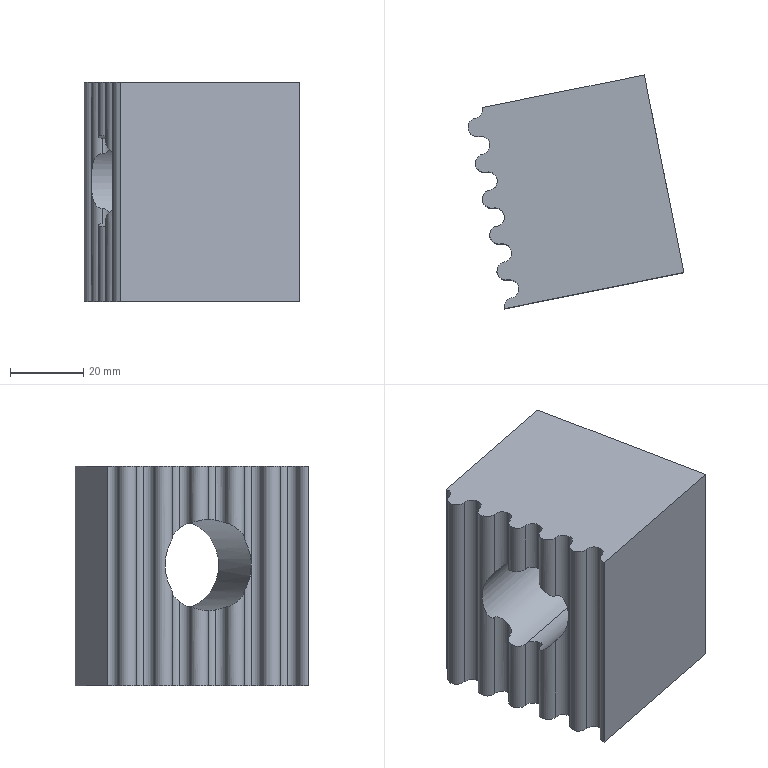Component | SolidWorks | ZTDJ-L-400-04-26-MaterialPortBagClamp-BagClampingAluminumBlock-1 | 1 solid | 47 faces | box 58.92 x 63.78 x 60 mm | volume 132216 mm3 | cylinder 34 | cone 8 | plane 5 | commonest cylinder face diameters 5 x32 25 x2 | material 6061-T6 (SS)
build123d program:
from build123d import *

# Parameters (mm, degrees)
SKETCH1_W             = 47.5
SKETCH1_H             = 55
BOSS_EXTRUDE1_DEPTH   = 30
SKETCH2_R             = 2.5
CUT_EXTRUDE1_DEPTH    = 71.145
SKETCH3_R             = 2.5
BOSS_EXTRUDE2_DEPTH   = 60
M6_TAPPED_HOLE1_D     = 5
M6_TAPPED_HOLE1_DEPTH = 15
M6_TAPPED_HOLE1_TIP   = 1.502
SKETCH6_R             = 12.5
CUT_EXTRUDE2_DEPTH    = 65.469


with BuildPart() as part:
    # Sketch1 → Boss-Extrude1 (new, symmetric)
    with BuildSketch(Plane.XY):
        Rectangle(SKETCH1_W, SKETCH1_H)
    extrude(amount=BOSS_EXTRUDE1_DEPTH, both=True)

    # Sketch2 → Cut-Extrude1 (cut, through all)
    with BuildSketch(Plane.XY.offset(30)):
        with Locations((-23.75, 22.5)):
            Circle(SKETCH2_R)
        with Locations((-23.75, 12.5)):
            Circle(SKETCH2_R)
        with Locations((-23.75, 2.5)):
            Circle(SKETCH2_R)
        with Locations((-23.75, -7.5)):
            Circle(SKETCH2_R)
        with Locations((-23.75, -17.5)):
            Circle(SKETCH2_R)
        with Locations((-23.75, -27.5)):
            Circle(SKETCH2_R)
    extrude(amount=-CUT_EXTRUDE1_DEPTH, mode=Mode.SUBTRACT)

    # Sketch3 → Boss-Extrude2 (add)
    with BuildSketch(Plane.XY.offset(30)):
        with Locations((-23.75, 17.5)):
            Circle(SKETCH3_R)
        with Locations((-23.75, 7.5)):
            Circle(SKETCH3_R)
        with Locations((-23.75, -2.5)):
            Circle(SKETCH3_R)
        with Locations((-23.75, -12.5)):
            Circle(SKETCH3_R)
        with Locations((-23.75, -22.5)):
            Circle(SKETCH3_R)
        with BuildLine():
            Line((-21.25, 27.5), (-26.25, 27.5))
            ThreePointArc((-26.25, 27.5), (-23.75, 25), (-21.25, 27.5))
        make_face()
    extrude(amount=-BOSS_EXTRUDE2_DEPTH)

    # M6 Tapped Hole1
    with Locations(Plane(origin=(23.75, 0, 0), x_dir=(0, 0, -1), z_dir=(1, 0, 0))):
        with Locations((-12, 15), (18, 15), (18, -15), (-12, -15)):
            Hole(M6_TAPPED_HOLE1_D / 2, depth=M6_TAPPED_HOLE1_DEPTH)
            with Locations((0, 0, -(M6_TAPPED_HOLE1_DEPTH + M6_TAPPED_HOLE1_TIP / 2))):  # 118° drill point
                Cone(0, M6_TAPPED_HOLE1_D / 2, M6_TAPPED_HOLE1_TIP, mode=Mode.SUBTRACT)

    # Sketch6 → Cut-Extrude2 (cut, through all)
    with BuildSketch(Plane(origin=(23.75, 0, 0), x_dir=(0, 0, -1), z_dir=(1, 0, 0))):
        with Locations((3, 0)):
            Circle(SKETCH6_R)
    extrude(amount=-CUT_EXTRUDE2_DEPTH, mode=Mode.SUBTRACT)


solid = part.part

# Placed as in the assembly
solid = solid.moved(Location((15.239, -186.918, 287), (180, 0, -11.367)))